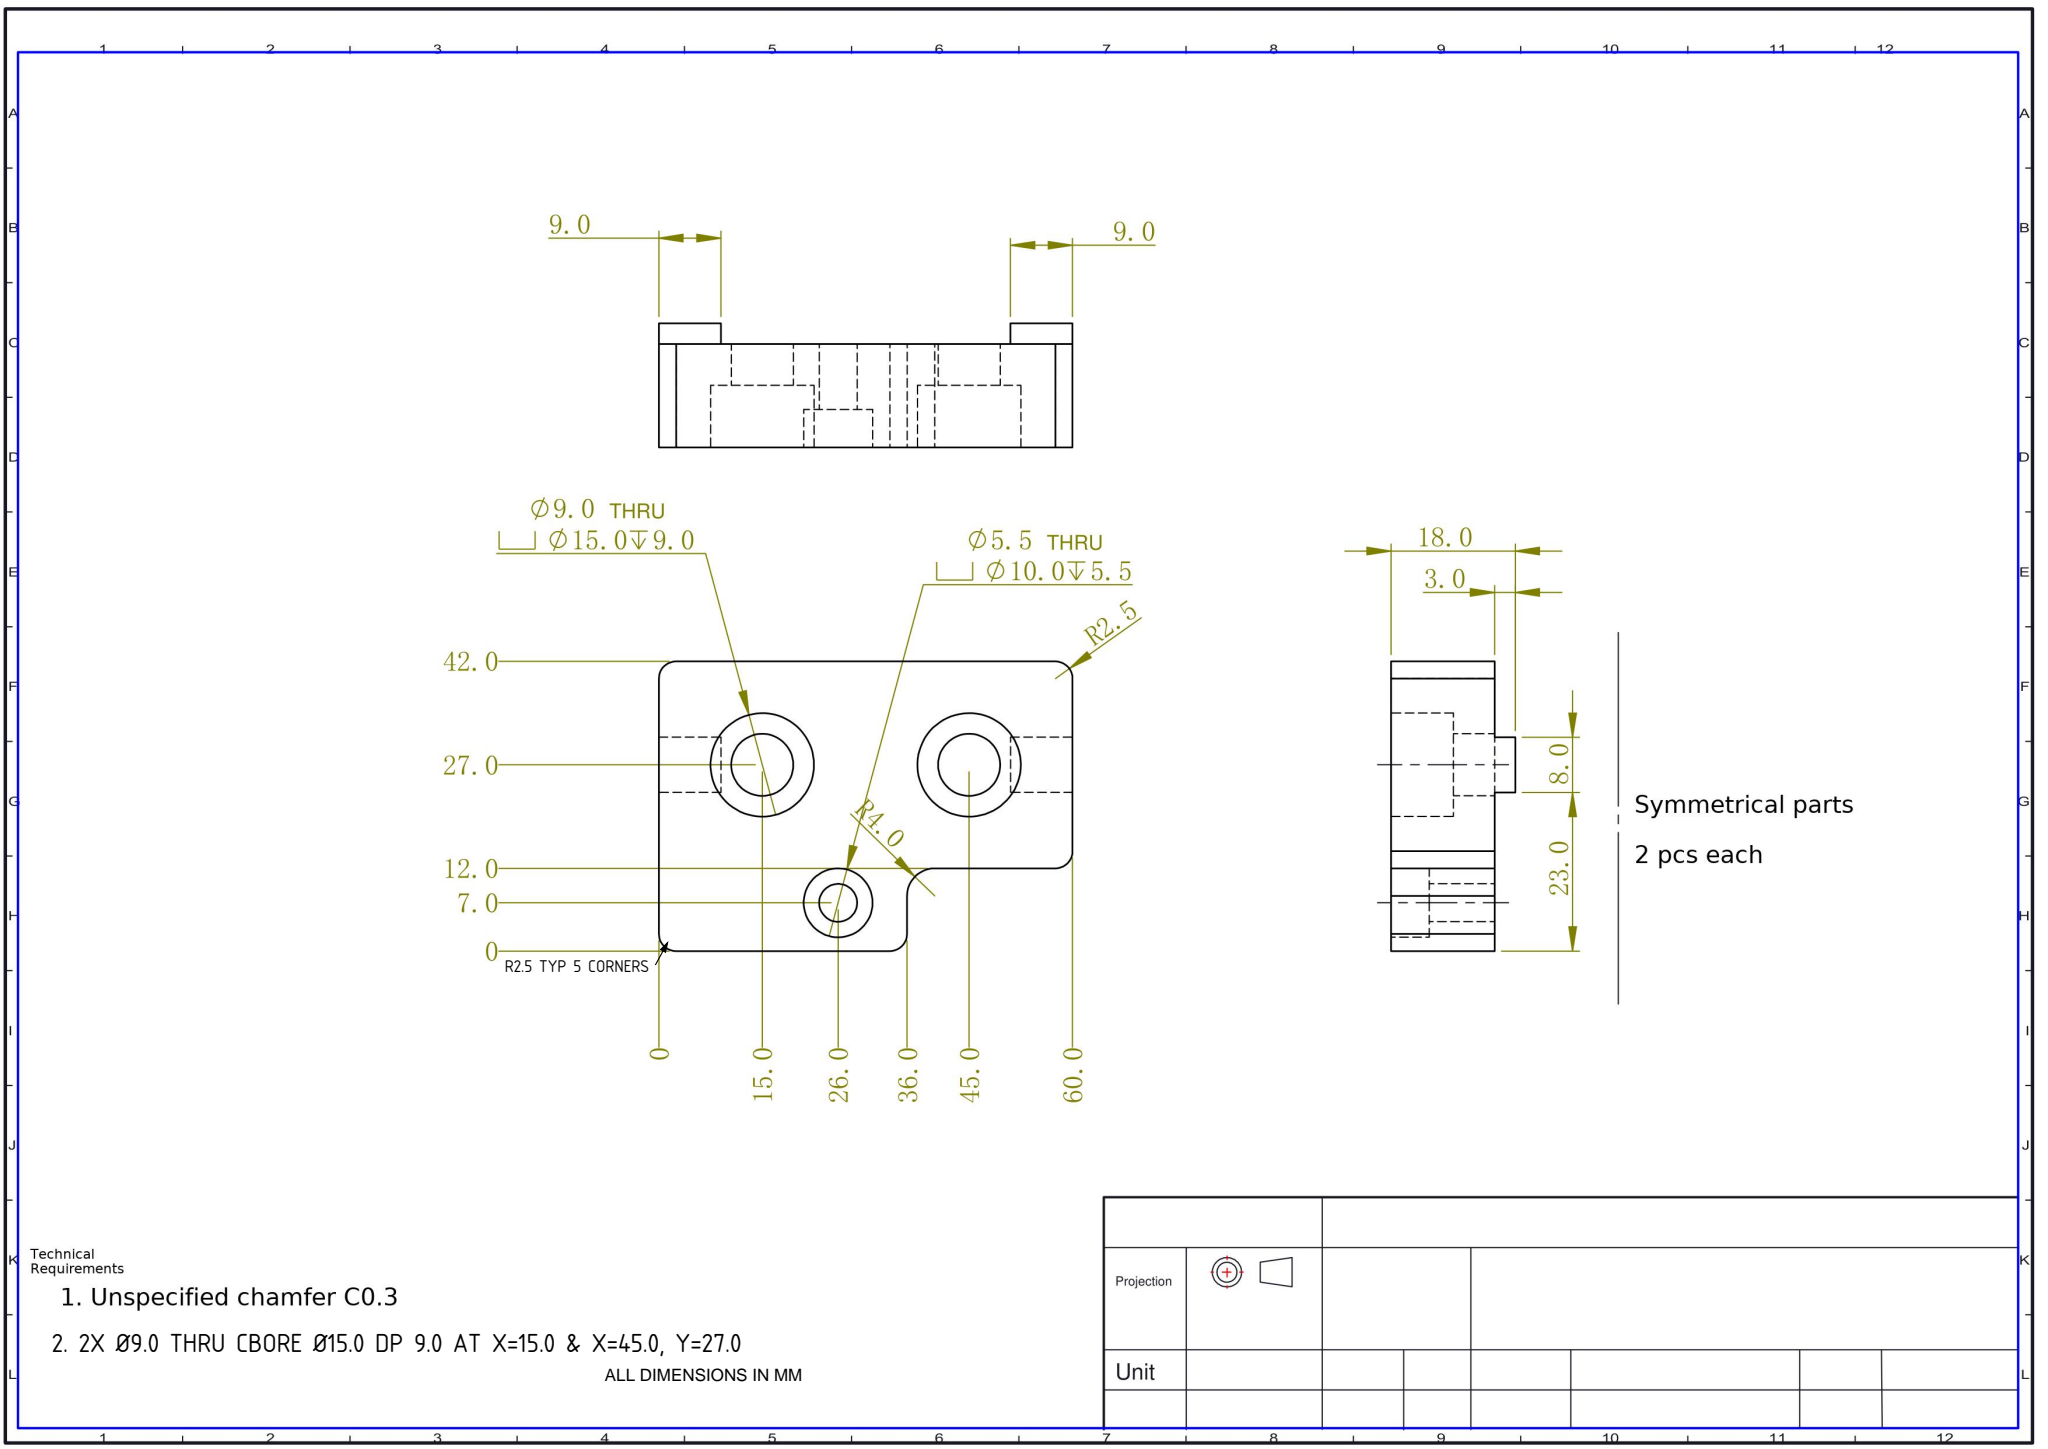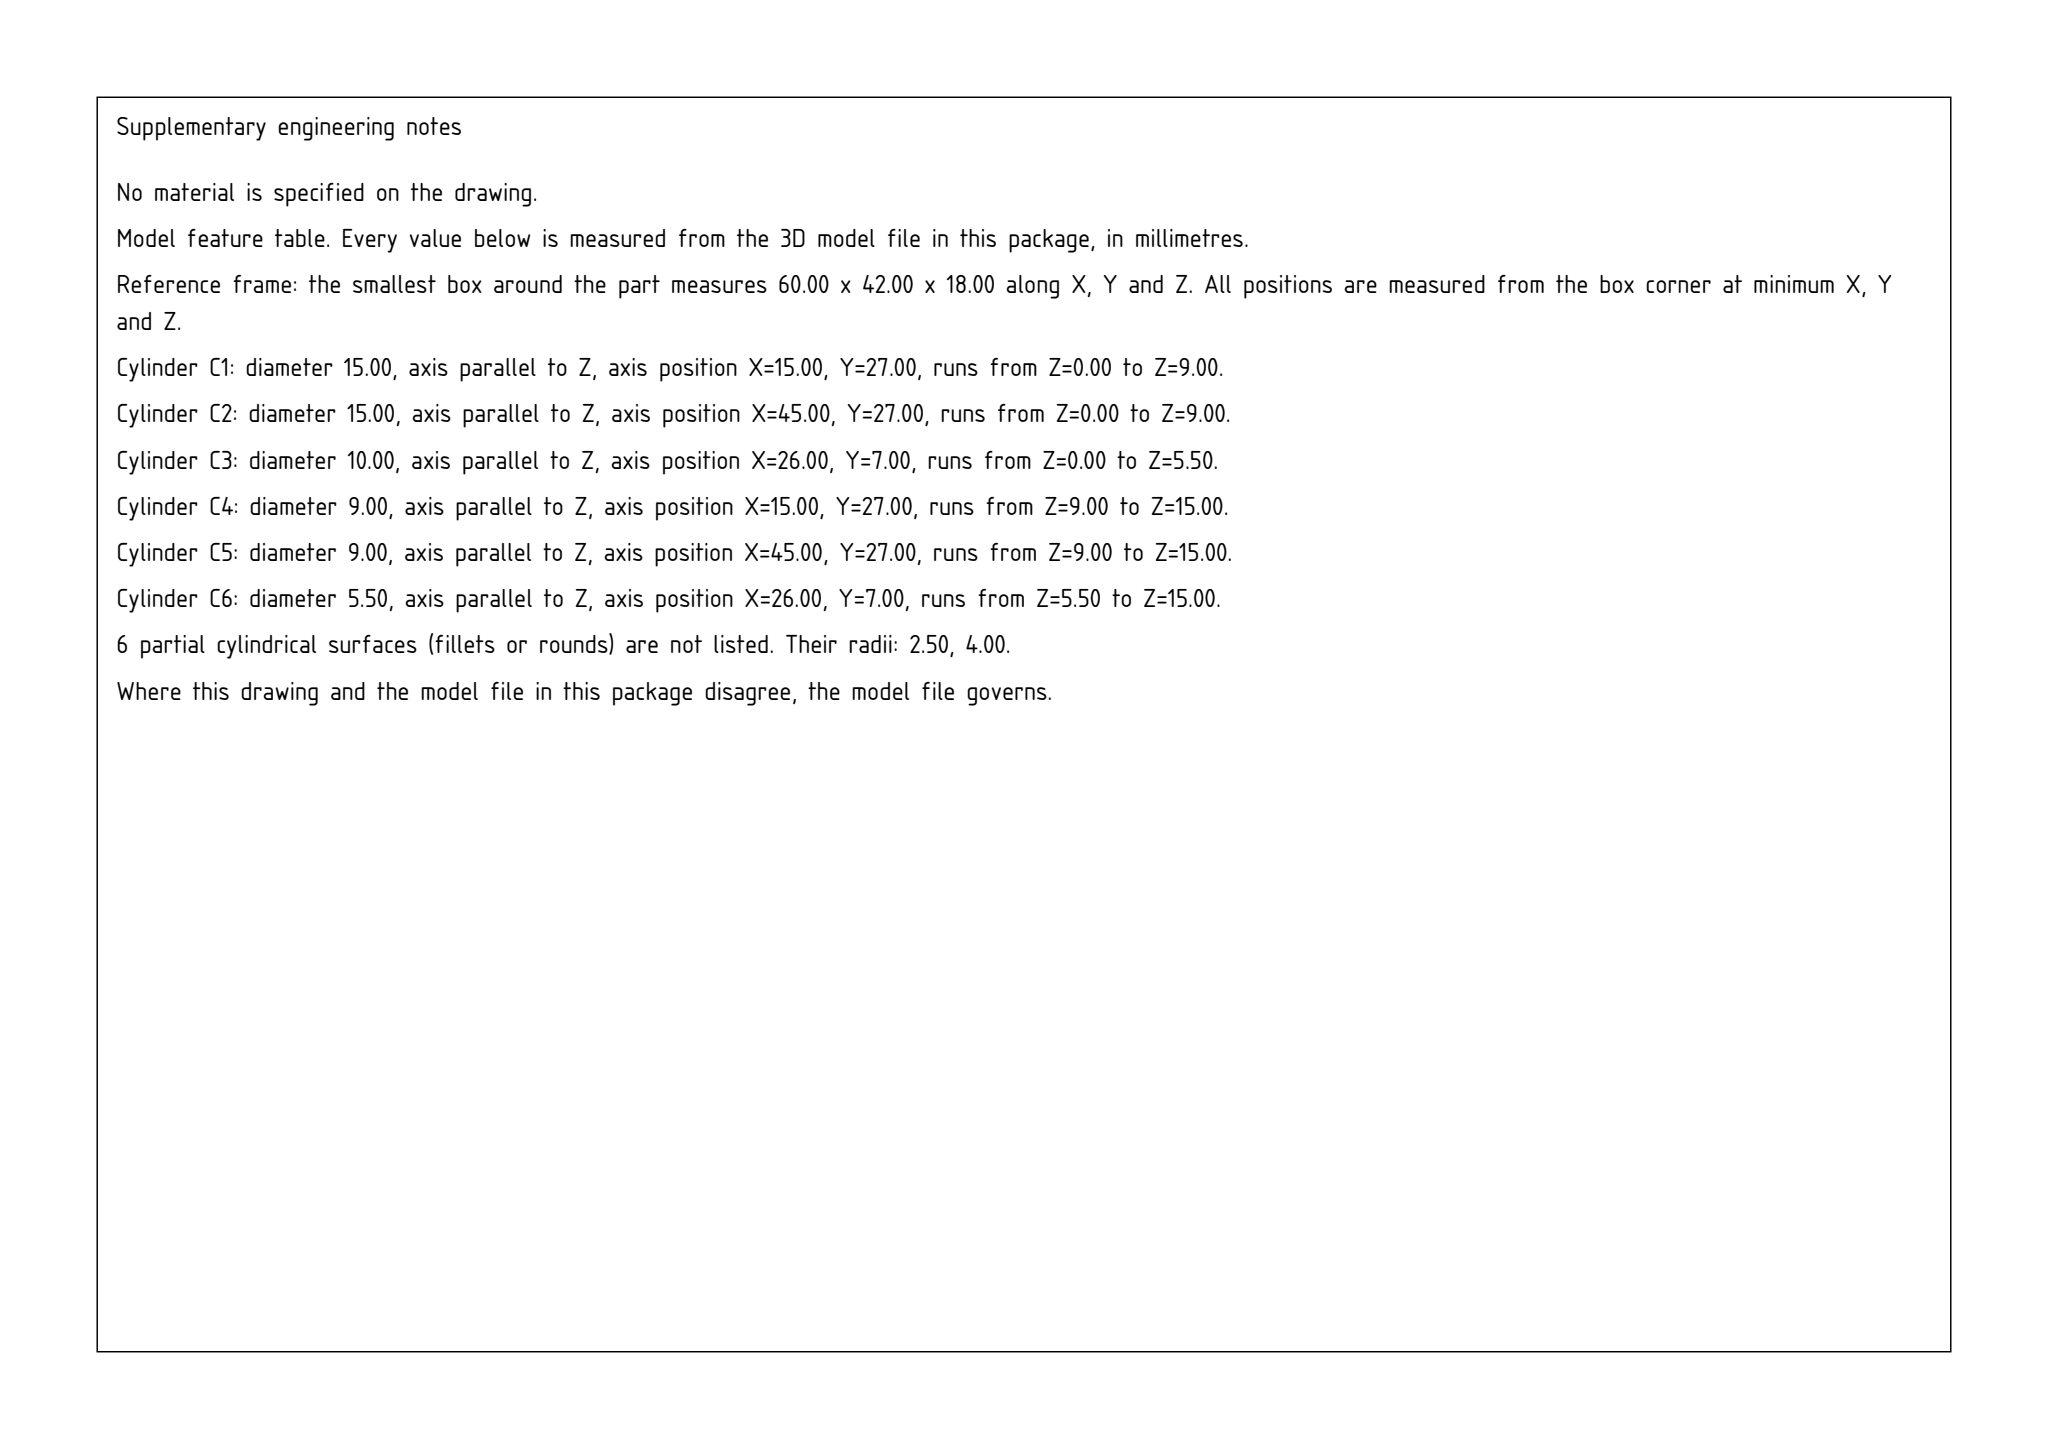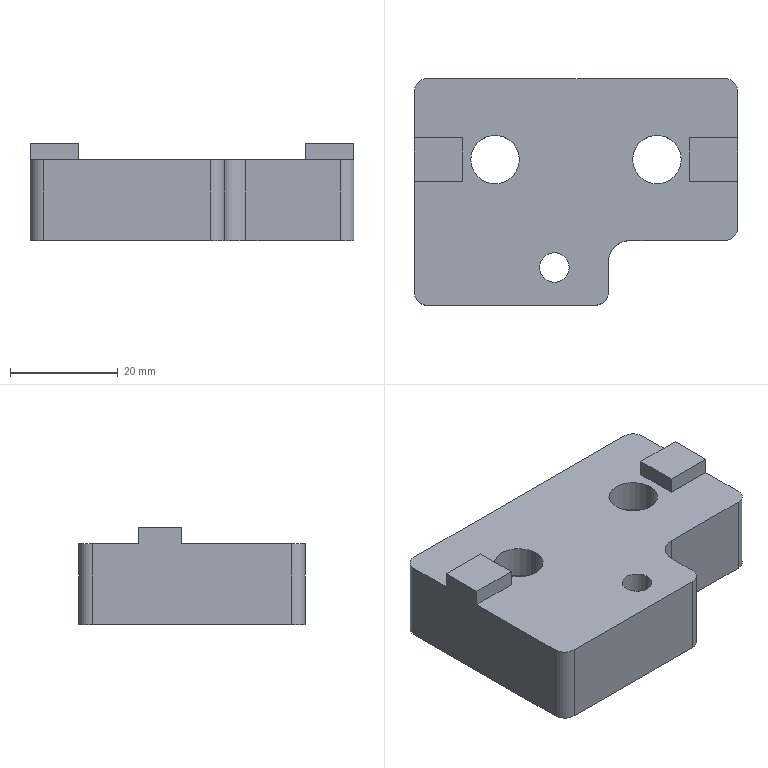Part | SolidWorks | mm | material S45C | 1 solid | 37 faces | box 60 x 42 x 18 mm | volume 29261 mm3 | plane 19 | cylinder 18 | commonest cylinder face diameters 5 x5 15 x4 9 x4 10 x2 5.5 x2 8 x1
Drawing notes:
2X Ø9.0 THRU CBORE Ø15.0 DP 9.0 AT X=15.0 & X=45.0, Y=27.0 | from the solid: Ø9.0 z-cyl at (15,27) & (45,27) L6.0 thru; Ø15.0 z-cyl same centers L9.0 counterbore
R2.5 TYP 5 OUTLINE CORNERS (NOTCH R4.0 EXCEPTED) | from the solid: Ø5.0 z-cyl corner rounds at (2.5,2.5),(2.5,39.5),(33.5,2.5),(57.5,14.5),(57.5,39.5) = R2.5